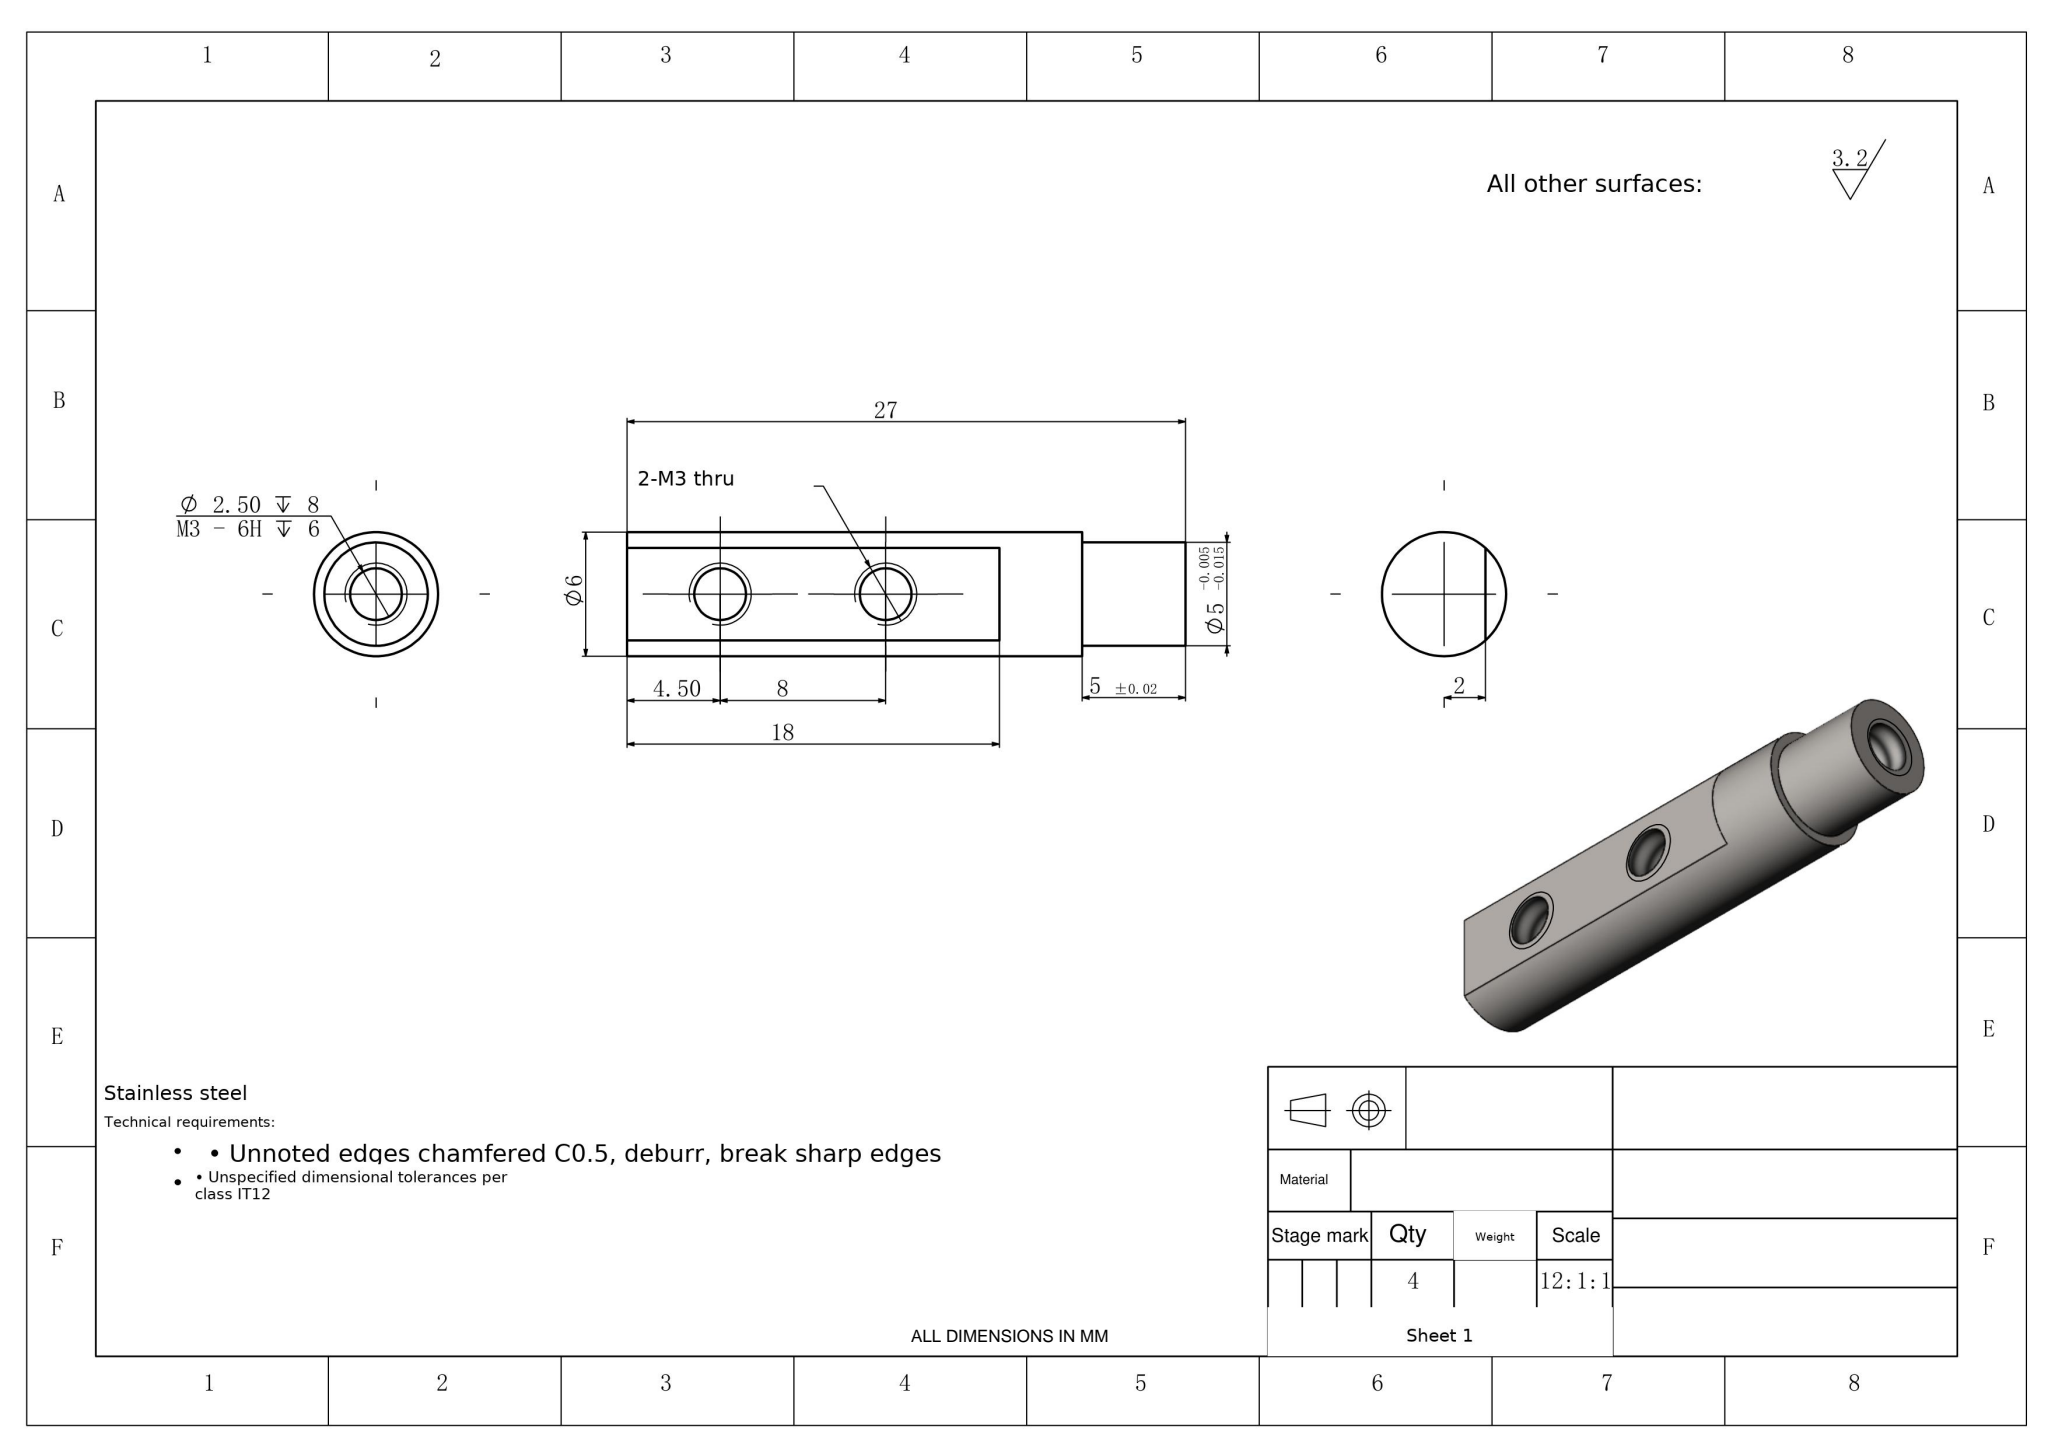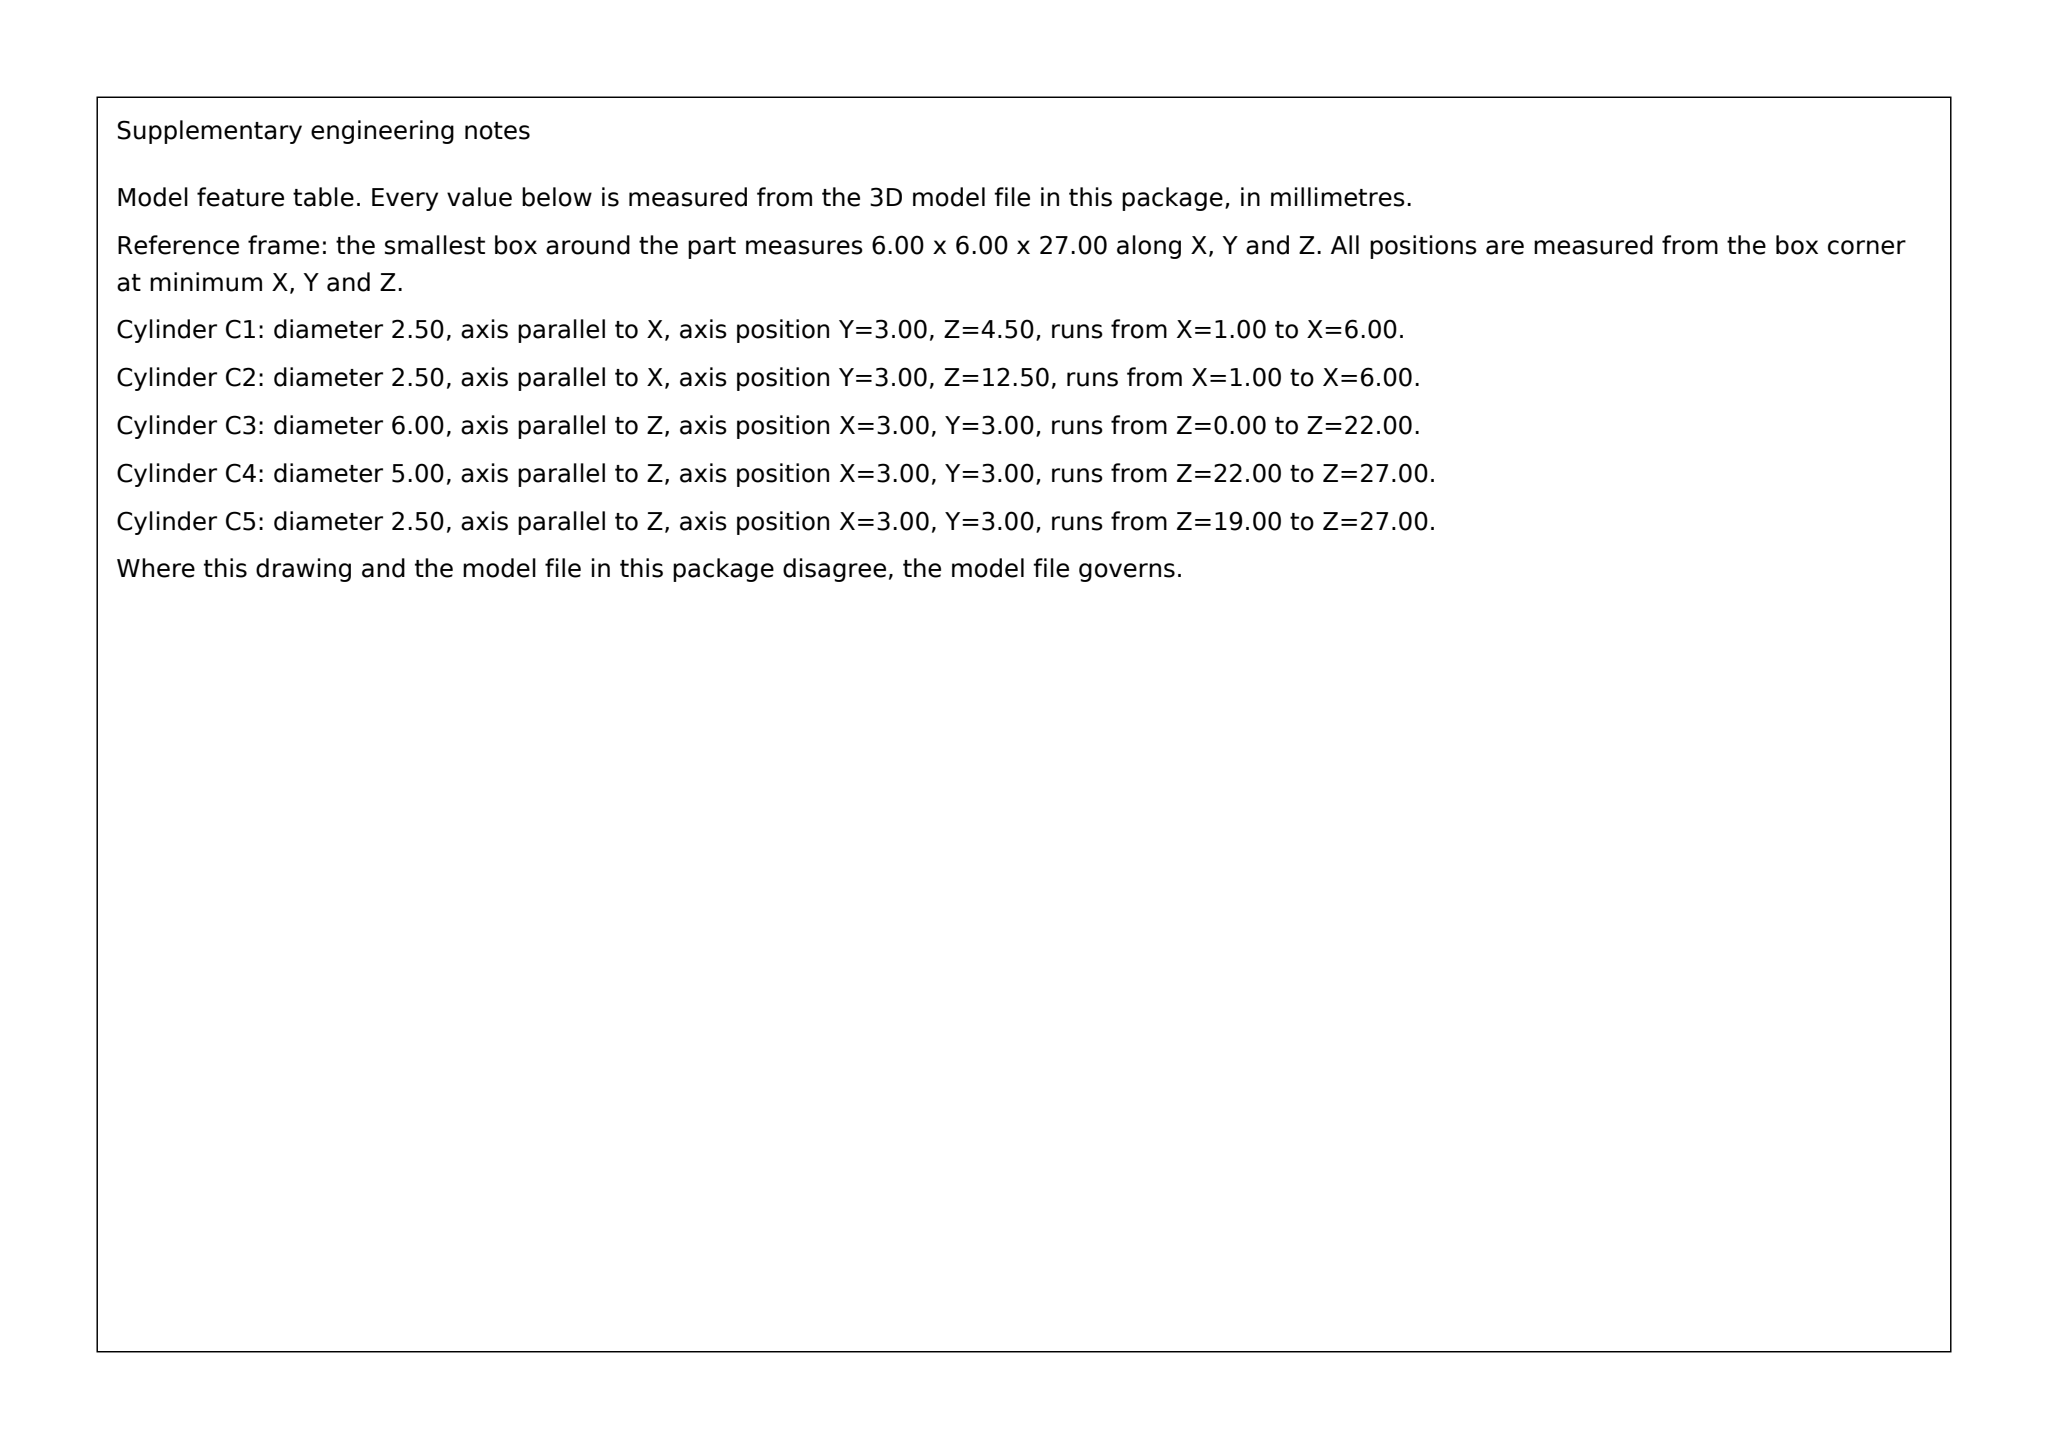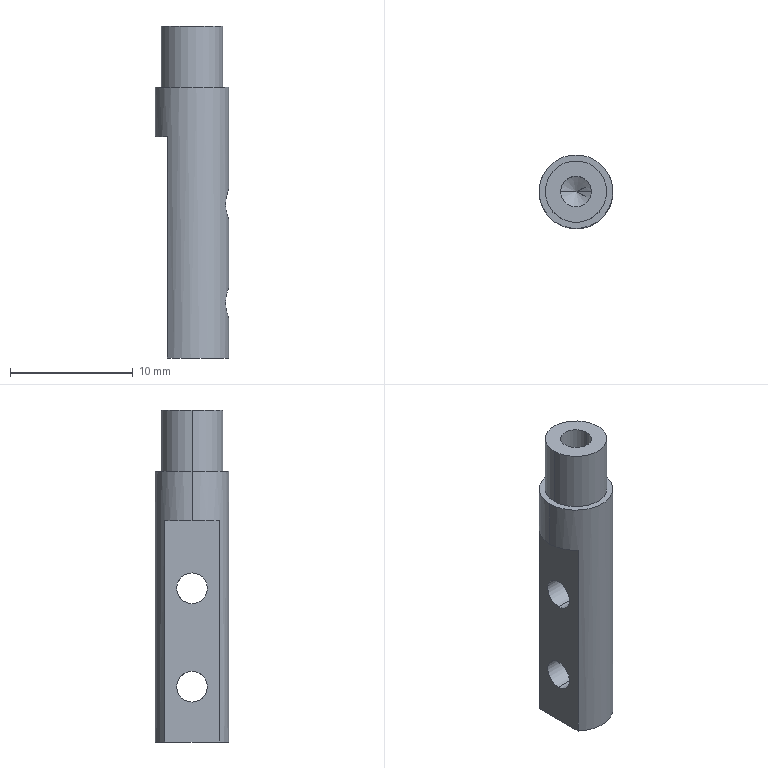Part | SolidWorks | mm | material Stainless steel | 1 solid | 17 faces | box 6 x 6 x 27 mm | volume 576 mm3 | cylinder 10 | plane 5 | cone 2 | commonest cylinder face diameters 2.5 x6 6 x2 5 x2
build123d program:
from build123d import *

# Parameters (mm, degrees)
SKETCH1_R             = 3
BOSS_EXTRUDE1_DEPTH   = 27
SKETCH2_W             = 4.131
SKETCH2_H             = 12.303
CUT_EXTRUDE1_DEPTH    = 18
M3_TAPPED_HOLE3_D     = 2.5
M3_TAPPED_HOLE2_D     = 2.5
M3_TAPPED_HOLE2_DEPTH = 8
M3_TAPPED_HOLE2_TIP   = 0.7511
SKETCH7_R             = 4.398
SKETCH7_R_2           = 2.5
CUT_EXTRUDE2_DEPTH    = 5


with BuildPart() as part:
    # Sketch1 → Boss-Extrude1 (new body)
    with BuildSketch(Plane.XY):
        Circle(SKETCH1_R)
    extrude(amount=BOSS_EXTRUDE1_DEPTH)

    # Sketch2 → Cut-Extrude1 (cut)
    with BuildSketch(Plane(origin=(0, 0, 0), x_dir=(-1, 0, 0), z_dir=(0, 0, -1))):
        with Locations((4.065, -2.134)):
            Rectangle(SKETCH2_W, SKETCH2_H)
    extrude(amount=-CUT_EXTRUDE1_DEPTH, mode=Mode.SUBTRACT)

    # M3 Tapped Hole3 (through all)
    with Locations(Plane.ZY.offset(2)):
        with Locations((12.5, 0), (4.5, 0)):
            Hole(M3_TAPPED_HOLE3_D / 2)

    # M3 Tapped Hole2
    with Locations(Plane.XY.offset(27)):
        with Locations((0, 0)):
            Hole(M3_TAPPED_HOLE2_D / 2, depth=M3_TAPPED_HOLE2_DEPTH)
            with Locations((0, 0, -(M3_TAPPED_HOLE2_DEPTH + M3_TAPPED_HOLE2_TIP / 2))):  # 118° drill point
                Cone(0, M3_TAPPED_HOLE2_D / 2, M3_TAPPED_HOLE2_TIP, mode=Mode.SUBTRACT)

    # Sketch7 → Cut-Extrude2 (cut)
    with BuildSketch(Plane.XY.offset(27)):
        Circle(SKETCH7_R)
        Circle(SKETCH7_R_2, mode=Mode.SUBTRACT)
    extrude(amount=-CUT_EXTRUDE2_DEPTH, mode=Mode.SUBTRACT)


solid = part.part
STEP:
#1=CARTESIAN_POINT('',(3.,0.,22.));
#2=VERTEX_POINT('',#1);
#3=CARTESIAN_POINT('',(-3.,0.,22.));
#4=VERTEX_POINT('',#3);
#5=CARTESIAN_POINT('',(0.,0.,22.));
#6=DIRECTION('',(0.,0.,1.));
#7=DIRECTION('',(1.,0.,0.));
#8=AXIS2_PLACEMENT_3D('',#5,#6,#7);
#9=CIRCLE('',#8,3.);
#10=EDGE_CURVE('',#2,#4,#9,.T.);
#11=ORIENTED_EDGE('',*,*,#10,.F.);
#12=CARTESIAN_POINT('',(3.,0.,13.75));
#13=VERTEX_POINT('',#12);
#14=CARTESIAN_POINT('',(3.,0.,27.));
#15=DIRECTION('',(0.,0.,-1.));
#16=VECTOR('',#15,1000.);
#17=LINE('',#14,#16);
#18=EDGE_CURVE('',#2,#13,#17,.T.);
#19=ORIENTED_EDGE('',*,*,#18,.T.);
#20=CARTESIAN_POINT('',(3.,0.,11.25));
#21=VERTEX_POINT('',#20);
#22=CARTESIAN_POINT('',(3.,0.,13.75));
#23=CARTESIAN_POINT('',(3.,0.08362,13.75));
#24=CARTESIAN_POINT('',(2.997,0.1657,13.742));
#25=CARTESIAN_POINT('',(2.983,0.3268,13.709));
#26=CARTESIAN_POINT('',(2.973,0.4067,13.685));
#27=CARTESIAN_POINT('',(2.936,0.6333,13.59));
#28=CARTESIAN_POINT('',(2.902,0.7706,13.497));
#29=CARTESIAN_POINT('',(2.832,0.9984,13.269));
#30=CARTESIAN_POINT('',(2.795,1.091,13.132));
#31=CARTESIAN_POINT('',(2.743,1.216,12.832));
#32=CARTESIAN_POINT('',(2.727,1.25,12.666));
#33=CARTESIAN_POINT('',(2.727,1.25,12.418));
#34=CARTESIAN_POINT('',(2.731,1.242,12.334));
#35=CARTESIAN_POINT('',(2.746,1.209,12.173));
#36=CARTESIAN_POINT('',(2.756,1.185,12.094));
#37=CARTESIAN_POINT('',(2.796,1.09,11.866));
#38=CARTESIAN_POINT('',(2.832,0.9979,11.73));
#39=CARTESIAN_POINT('',(2.902,0.7693,11.502));
#40=CARTESIAN_POINT('',(2.937,0.6315,11.409));
#41=CARTESIAN_POINT('',(2.986,0.3311,11.284));
#42=CARTESIAN_POINT('',(3.,0.1647,11.25));
#43=CARTESIAN_POINT('',(3.,0.,11.25));
#44=B_SPLINE_CURVE_WITH_KNOTS('',3,(#22,#23,#24,#25,#26,#27,#28,#29,#30,#31,#32,#33,#34,#35,#36,#37,#38,#39,#40,#41,#42,#43),.UNSPECIFIED.,.F.,.F.,(4,2,2,2,2,2,2,2,2,2,4),(0.,0.0002471,0.0004942,0.0009884,0.001483,0.001977,0.002224,0.002471,0.002965,0.003459,0.003954),.UNSPECIFIED.);
#45=EDGE_CURVE('',#13,#21,#44,.T.);
#46=ORIENTED_EDGE('',*,*,#45,.T.);
#47=CARTESIAN_POINT('',(3.,0.,5.75));
#48=VERTEX_POINT('',#47);
#49=CARTESIAN_POINT('',(3.,0.,27.));
#50=DIRECTION('',(0.,0.,-1.));
#51=VECTOR('',#50,1000.);
#52=LINE('',#49,#51);
#53=EDGE_CURVE('',#21,#48,#52,.T.);
#54=ORIENTED_EDGE('',*,*,#53,.T.);
#55=CARTESIAN_POINT('',(3.,0.,3.25));
#56=VERTEX_POINT('',#55);
#57=CARTESIAN_POINT('',(3.,0.,5.75));
#58=CARTESIAN_POINT('',(3.,0.08362,5.75));
#59=CARTESIAN_POINT('',(2.997,0.1657,5.742));
#60=CARTESIAN_POINT('',(2.983,0.3268,5.709));
#61=CARTESIAN_POINT('',(2.973,0.4067,5.685));
#62=CARTESIAN_POINT('',(2.936,0.6333,5.59));
#63=CARTESIAN_POINT('',(2.902,0.7706,5.497));
#64=CARTESIAN_POINT('',(2.832,0.9984,5.269));
#65=CARTESIAN_POINT('',(2.795,1.091,5.132));
#66=CARTESIAN_POINT('',(2.743,1.216,4.832));
#67=CARTESIAN_POINT('',(2.727,1.25,4.666));
#68=CARTESIAN_POINT('',(2.727,1.25,4.418));
#69=CARTESIAN_POINT('',(2.731,1.242,4.334));
#70=CARTESIAN_POINT('',(2.746,1.209,4.173));
#71=CARTESIAN_POINT('',(2.756,1.185,4.094));
#72=CARTESIAN_POINT('',(2.796,1.09,3.866));
#73=CARTESIAN_POINT('',(2.832,0.9979,3.73));
#74=CARTESIAN_POINT('',(2.902,0.7693,3.502));
#75=CARTESIAN_POINT('',(2.937,0.6315,3.409));
#76=CARTESIAN_POINT('',(2.986,0.3311,3.284));
#77=CARTESIAN_POINT('',(3.,0.1647,3.25));
#78=CARTESIAN_POINT('',(3.,0.,3.25));
#79=B_SPLINE_CURVE_WITH_KNOTS('',3,(#57,#58,#59,#60,#61,#62,#63,#64,#65,#66,#67,#68,#69,#70,#71,#72,#73,#74,#75,#76,#77,#78),.UNSPECIFIED.,.F.,.F.,(4,2,2,2,2,2,2,2,2,2,4),(0.,0.0002471,0.0004942,0.0009884,0.001483,0.001977,0.002224,0.002471,0.002965,0.003459,0.003954),.UNSPECIFIED.);
#80=EDGE_CURVE('',#48,#56,#79,.T.);
#81=ORIENTED_EDGE('',*,*,#80,.T.);
#82=CARTESIAN_POINT('',(3.,0.,0.));
#83=VERTEX_POINT('',#82);
#84=CARTESIAN_POINT('',(3.,0.,27.));
#85=DIRECTION('',(0.,0.,-1.));
#86=VECTOR('',#85,1000.);
#87=LINE('',#84,#86);
#88=EDGE_CURVE('',#56,#83,#87,.T.);
#89=ORIENTED_EDGE('',*,*,#88,.T.);
#90=CARTESIAN_POINT('',(-2.,2.236,0.));
#91=VERTEX_POINT('',#90);
#92=CARTESIAN_POINT('',(0.,0.,0.));
#93=DIRECTION('',(0.,0.,1.));
#94=DIRECTION('',(1.,0.,0.));
#95=AXIS2_PLACEMENT_3D('',#92,#93,#94);
#96=CIRCLE('',#95,3.);
#97=EDGE_CURVE('',#83,#91,#96,.T.);
#98=ORIENTED_EDGE('',*,*,#97,.T.);
#99=CARTESIAN_POINT('',(-2.,2.236,18.));
#100=VERTEX_POINT('',#99);
#101=CARTESIAN_POINT('',(-2.,2.236,27.));
#102=DIRECTION('',(0.,0.,1.));
#103=VECTOR('',#102,1000.);
#104=LINE('',#101,#103);
#105=EDGE_CURVE('',#91,#100,#104,.T.);
#106=ORIENTED_EDGE('',*,*,#105,.T.);
#107=CARTESIAN_POINT('',(-3.,0.,18.));
#108=VERTEX_POINT('',#107);
#109=CARTESIAN_POINT('',(0.,0.,18.));
#110=DIRECTION('',(0.,0.,1.));
#111=DIRECTION('',(1.,0.,0.));
#112=AXIS2_PLACEMENT_3D('',#109,#110,#111);
#113=CIRCLE('',#112,3.);
#114=EDGE_CURVE('',#100,#108,#113,.T.);
#115=ORIENTED_EDGE('',*,*,#114,.T.);
#116=CARTESIAN_POINT('',(-3.,0.,27.));
#117=DIRECTION('',(0.,0.,-1.));
#118=VECTOR('',#117,1000.);
#119=LINE('',#116,#118);
#120=EDGE_CURVE('',#4,#108,#119,.T.);
#121=ORIENTED_EDGE('',*,*,#120,.F.);
#122=EDGE_LOOP('',(#11,#19,#46,#54,#81,#89,#98,#106,#115,#121));
#123=FACE_OUTER_BOUND('',#122,.T.);
#124=CARTESIAN_POINT('',(0.,0.,27.));
#125=DIRECTION('',(0.,0.,-1.));
#126=DIRECTION('',(-1.,0.,0.));
#127=AXIS2_PLACEMENT_3D('',#124,#125,#126);
#128=CYLINDRICAL_SURFACE('',#127,3.);
#129=ADVANCED_FACE('',(#123),#128,.T.);
#130=CARTESIAN_POINT('',(3.,0.,3.25));
#131=CARTESIAN_POINT('',(3.,-0.1646,3.25));
#132=CARTESIAN_POINT('',(2.986,-0.3304,3.283));
#133=CARTESIAN_POINT('',(2.936,-0.6331,3.41));
#134=CARTESIAN_POINT('',(2.902,-0.7697,3.502));
#135=CARTESIAN_POINT('',(2.849,-0.9421,3.674));
#136=CARTESIAN_POINT('',(2.831,-0.9932,3.737));
#137=CARTESIAN_POINT('',(2.798,-1.083,3.871));
#138=CARTESIAN_POINT('',(2.782,-1.122,3.944));
#139=CARTESIAN_POINT('',(2.756,-1.185,4.094));
#140=CARTESIAN_POINT('',(2.746,-1.209,4.172));
#141=CARTESIAN_POINT('',(2.731,-1.242,4.333));
#142=CARTESIAN_POINT('',(2.727,-1.25,4.417));
#143=CARTESIAN_POINT('',(2.727,-1.25,4.664));
#144=CARTESIAN_POINT('',(2.743,-1.217,4.83));
#145=CARTESIAN_POINT('',(2.795,-1.091,5.132));
#146=CARTESIAN_POINT('',(2.831,-0.9991,5.269));
#147=CARTESIAN_POINT('',(2.902,-0.7697,5.498));
#148=CARTESIAN_POINT('',(2.936,-0.6344,5.59));
#149=CARTESIAN_POINT('',(2.986,-0.3296,5.717));
#150=CARTESIAN_POINT('',(3.,-0.1671,5.75));
#151=CARTESIAN_POINT('',(3.,0.,5.75));
#152=B_SPLINE_CURVE_WITH_KNOTS('',3,(#130,#131,#132,#133,#134,#135,#136,#137,#138,#139,#140,#141,#142,#143,#144,#145,#146,#147,#148,#149,#150,#151),.UNSPECIFIED.,.F.,.F.,(4,2,2,2,2,2,2,2,2,2,4),(0.003954,0.004448,0.004941,0.005188,0.005435,0.005682,0.005929,0.006423,0.006917,0.00741,0.007904),.UNSPECIFIED.);
#153=EDGE_CURVE('',#56,#48,#152,.T.);
#154=ORIENTED_EDGE('',*,*,#153,.F.);
#155=CARTESIAN_POINT('',(-2.,0.,3.25));
#156=VERTEX_POINT('',#155);
#157=CARTESIAN_POINT('',(-2.,0.,3.25));
#158=DIRECTION('',(-1.,0.,0.));
#159=VECTOR('',#158,1000.);
#160=LINE('',#157,#159);
#161=EDGE_CURVE('',#56,#156,#160,.T.);
#162=ORIENTED_EDGE('',*,*,#161,.T.);
#163=CARTESIAN_POINT('',(-2.,0.,5.75));
#164=VERTEX_POINT('',#163);
#165=CARTESIAN_POINT('',(-2.,0.,4.5));
#166=DIRECTION('',(-1.,0.,0.));
#167=DIRECTION('',(0.,0.,1.));
#168=AXIS2_PLACEMENT_3D('',#165,#166,#167);
#169=CIRCLE('',#168,1.25);
#170=EDGE_CURVE('',#156,#164,#169,.T.);
#171=ORIENTED_EDGE('',*,*,#170,.T.);
#172=CARTESIAN_POINT('',(-2.,0.,5.75));
#173=DIRECTION('',(-1.,0.,0.));
#174=VECTOR('',#173,1000.);
#175=LINE('',#172,#174);
#176=EDGE_CURVE('',#48,#164,#175,.T.);
#177=ORIENTED_EDGE('',*,*,#176,.F.);
#178=EDGE_LOOP('',(#154,#162,#171,#177));
#179=FACE_OUTER_BOUND('',#178,.T.);
#180=CARTESIAN_POINT('',(-2.,0.,4.5));
#181=DIRECTION('',(-1.,0.,0.));
#182=DIRECTION('',(0.,0.,1.));
#183=AXIS2_PLACEMENT_3D('',#180,#181,#182);
#184=CYLINDRICAL_SURFACE('',#183,1.25);
#185=ADVANCED_FACE('',(#179),#184,.F.);
#186=CARTESIAN_POINT('',(3.,0.,11.25));
#187=CARTESIAN_POINT('',(3.,-0.1646,11.25));
#188=CARTESIAN_POINT('',(2.986,-0.3304,11.283));
#189=CARTESIAN_POINT('',(2.936,-0.6331,11.41));
#190=CARTESIAN_POINT('',(2.902,-0.7697,11.502));
#191=CARTESIAN_POINT('',(2.849,-0.9421,11.674));
#192=CARTESIAN_POINT('',(2.831,-0.9932,11.737));
#193=CARTESIAN_POINT('',(2.798,-1.083,11.871));
#194=CARTESIAN_POINT('',(2.782,-1.122,11.944));
#195=CARTESIAN_POINT('',(2.756,-1.185,12.094));
#196=CARTESIAN_POINT('',(2.746,-1.209,12.172));
#197=CARTESIAN_POINT('',(2.731,-1.242,12.333));
#198=CARTESIAN_POINT('',(2.727,-1.25,12.417));
#199=CARTESIAN_POINT('',(2.727,-1.25,12.664));
#200=CARTESIAN_POINT('',(2.743,-1.217,12.83));
#201=CARTESIAN_POINT('',(2.795,-1.091,13.132));
#202=CARTESIAN_POINT('',(2.831,-0.9991,13.269));
#203=CARTESIAN_POINT('',(2.902,-0.7697,13.498));
#204=CARTESIAN_POINT('',(2.936,-0.6344,13.59));
#205=CARTESIAN_POINT('',(2.986,-0.3296,13.717));
#206=CARTESIAN_POINT('',(3.,-0.1671,13.75));
#207=CARTESIAN_POINT('',(3.,0.,13.75));
#208=B_SPLINE_CURVE_WITH_KNOTS('',3,(#186,#187,#188,#189,#190,#191,#192,#193,#194,#195,#196,#197,#198,#199,#200,#201,#202,#203,#204,#205,#206,#207),.UNSPECIFIED.,.F.,.F.,(4,2,2,2,2,2,2,2,2,2,4),(0.003954,0.004448,0.004941,0.005188,0.005435,0.005682,0.005929,0.006423,0.006917,0.00741,0.007904),.UNSPECIFIED.);
#209=EDGE_CURVE('',#21,#13,#208,.T.);
#210=ORIENTED_EDGE('',*,*,#209,.F.);
#211=CARTESIAN_POINT('',(-2.,0.,11.25));
#212=VERTEX_POINT('',#211);
#213=CARTESIAN_POINT('',(-2.,0.,11.25));
#214=DIRECTION('',(-1.,0.,0.));
#215=VECTOR('',#214,1000.);
#216=LINE('',#213,#215);
#217=EDGE_CURVE('',#21,#212,#216,.T.);
#218=ORIENTED_EDGE('',*,*,#217,.T.);
#219=CARTESIAN_POINT('',(-2.,0.,13.75));
#220=VERTEX_POINT('',#219);
#221=CARTESIAN_POINT('',(-2.,0.,12.5));
#222=DIRECTION('',(-1.,0.,0.));
#223=DIRECTION('',(0.,0.,1.));
#224=AXIS2_PLACEMENT_3D('',#221,#222,#223);
#225=CIRCLE('',#224,1.25);
#226=EDGE_CURVE('',#212,#220,#225,.T.);
#227=ORIENTED_EDGE('',*,*,#226,.T.);
#228=CARTESIAN_POINT('',(-2.,0.,13.75));
#229=DIRECTION('',(-1.,0.,0.));
#230=VECTOR('',#229,1000.);
#231=LINE('',#228,#230);
#232=EDGE_CURVE('',#13,#220,#231,.T.);
#233=ORIENTED_EDGE('',*,*,#232,.F.);
#234=EDGE_LOOP('',(#210,#218,#227,#233));
#235=FACE_OUTER_BOUND('',#234,.T.);
#236=CARTESIAN_POINT('',(-2.,0.,12.5));
#237=DIRECTION('',(-1.,0.,0.));
#238=DIRECTION('',(0.,0.,1.));
#239=AXIS2_PLACEMENT_3D('',#236,#237,#238);
#240=CYLINDRICAL_SURFACE('',#239,1.25);
#241=ADVANCED_FACE('',(#235),#240,.F.);
#242=CARTESIAN_POINT('',(2.5,0.,22.));
#243=VERTEX_POINT('',#242);
#244=CARTESIAN_POINT('',(-2.5,0.,22.));
#245=VERTEX_POINT('',#244);
#246=CARTESIAN_POINT('',(0.,0.,22.));
#247=DIRECTION('',(0.,0.,1.));
#248=DIRECTION('',(1.,0.,0.));
#249=AXIS2_PLACEMENT_3D('',#246,#247,#248);
#250=CIRCLE('',#249,2.5);
#251=EDGE_CURVE('',#243,#245,#250,.T.);
#252=ORIENTED_EDGE('',*,*,#251,.T.);
#253=CARTESIAN_POINT('',(-2.5,0.,27.));
#254=VERTEX_POINT('',#253);
#255=CARTESIAN_POINT('',(-2.5,0.,22.));
#256=DIRECTION('',(0.,0.,1.));
#257=VECTOR('',#256,1000.);
#258=LINE('',#255,#257);
#259=EDGE_CURVE('',#245,#254,#258,.T.);
#260=ORIENTED_EDGE('',*,*,#259,.T.);
#261=CARTESIAN_POINT('',(2.5,0.,27.));
#262=VERTEX_POINT('',#261);
#263=CARTESIAN_POINT('',(0.,0.,27.));
#264=DIRECTION('',(0.,0.,1.));
#265=DIRECTION('',(1.,0.,0.));
#266=AXIS2_PLACEMENT_3D('',#263,#264,#265);
#267=CIRCLE('',#266,2.5);
#268=EDGE_CURVE('',#262,#254,#267,.T.);
#269=ORIENTED_EDGE('',*,*,#268,.F.);
#270=CARTESIAN_POINT('',(2.5,0.,22.));
#271=DIRECTION('',(0.,0.,1.));
#272=VECTOR('',#271,1000.);
#273=LINE('',#270,#272);
#274=EDGE_CURVE('',#243,#262,#273,.T.);
#275=ORIENTED_EDGE('',*,*,#274,.F.);
#276=EDGE_LOOP('',(#252,#260,#269,#275));
#277=FACE_OUTER_BOUND('',#276,.T.);
#278=CARTESIAN_POINT('',(0.,0.,22.));
#279=DIRECTION('',(0.,0.,1.));
#280=DIRECTION('',(1.,0.,0.));
#281=AXIS2_PLACEMENT_3D('',#278,#279,#280);
#282=CYLINDRICAL_SURFACE('',#281,2.5);
#283=ADVANCED_FACE('',(#277),#282,.T.);
#284=CARTESIAN_POINT('',(-1.25,0.,19.));
#285=VERTEX_POINT('',#284);
#286=CARTESIAN_POINT('',(1.25,0.,19.));
#287=VERTEX_POINT('',#286);
#288=CARTESIAN_POINT('',(0.,0.,19.));
#289=DIRECTION('',(0.,0.,1.));
#290=DIRECTION('',(1.,0.,0.));
#291=AXIS2_PLACEMENT_3D('',#288,#289,#290);
#292=CIRCLE('',#291,1.25);
#293=EDGE_CURVE('',#285,#287,#292,.T.);
#294=ORIENTED_EDGE('',*,*,#293,.F.);
#295=CARTESIAN_POINT('',(-1.25,0.,27.));
#296=VERTEX_POINT('',#295);
#297=CARTESIAN_POINT('',(-1.25,0.,27.));
#298=DIRECTION('',(0.,0.,1.));
#299=VECTOR('',#298,1000.);
#300=LINE('',#297,#299);
#301=EDGE_CURVE('',#285,#296,#300,.T.);
#302=ORIENTED_EDGE('',*,*,#301,.T.);
#303=CARTESIAN_POINT('',(1.25,0.,27.));
#304=VERTEX_POINT('',#303);
#305=CARTESIAN_POINT('',(0.,0.,27.));
#306=DIRECTION('',(0.,0.,1.));
#307=DIRECTION('',(1.,0.,0.));
#308=AXIS2_PLACEMENT_3D('',#305,#306,#307);
#309=CIRCLE('',#308,1.25);
#310=EDGE_CURVE('',#296,#304,#309,.T.);
#311=ORIENTED_EDGE('',*,*,#310,.T.);
#312=CARTESIAN_POINT('',(1.25,0.,27.));
#313=DIRECTION('',(0.,0.,1.));
#314=VECTOR('',#313,1000.);
#315=LINE('',#312,#314);
#316=EDGE_CURVE('',#287,#304,#315,.T.);
#317=ORIENTED_EDGE('',*,*,#316,.F.);
#318=EDGE_LOOP('',(#294,#302,#311,#317));
#319=FACE_OUTER_BOUND('',#318,.T.);
#320=CARTESIAN_POINT('',(0.,0.,27.));
#321=DIRECTION('',(0.,0.,1.));
#322=DIRECTION('',(1.,0.,0.));
#323=AXIS2_PLACEMENT_3D('',#320,#321,#322);
#324=CYLINDRICAL_SURFACE('',#323,1.25);
#325=ADVANCED_FACE('',(#319),#324,.F.);
#326=CARTESIAN_POINT('',(-0.,0.,18.249));
#327=VERTEX_POINT('',#326);
#328=CARTESIAN_POINT('',(1.25,0.,19.));
#329=DIRECTION('',(0.8572,0.,0.515));
#330=VECTOR('',#329,1000.);
#331=LINE('',#328,#330);
#332=EDGE_CURVE('',#327,#287,#331,.T.);
#333=ORIENTED_EDGE('',*,*,#332,.F.);
#334=CARTESIAN_POINT('',(-1.25,0.,19.));
#335=DIRECTION('',(-0.8572,0.,0.515));
#336=VECTOR('',#335,1000.);
#337=LINE('',#334,#336);
#338=EDGE_CURVE('',#327,#285,#337,.T.);
#339=ORIENTED_EDGE('',*,*,#338,.T.);
#340=ORIENTED_EDGE('',*,*,#293,.T.);
#341=EDGE_LOOP('',(#333,#339,#340));
#342=FACE_OUTER_BOUND('',#341,.T.);
#343=CARTESIAN_POINT('',(0.,0.,19.));
#344=DIRECTION('',(0.,0.,1.));
#345=DIRECTION('',(1.,0.,0.));
#346=AXIS2_PLACEMENT_3D('',#343,#344,#345);
#347=CONICAL_SURFACE('',#346,1.25,1.03);
#348=ADVANCED_FACE('',(#342),#347,.F.);
#349=CARTESIAN_POINT('',(0.,0.,27.));
#350=DIRECTION('',(0.,0.,1.));
#351=DIRECTION('',(1.,0.,0.));
#352=AXIS2_PLACEMENT_3D('',#349,#350,#351);
#353=CIRCLE('',#352,1.25);
#354=EDGE_CURVE('',#304,#296,#353,.T.);
#355=ORIENTED_EDGE('',*,*,#354,.F.);
#356=ORIENTED_EDGE('',*,*,#310,.F.);
#357=EDGE_LOOP('',(#355,#356));
#358=FACE_BOUND('',#357,.T.);
#359=ORIENTED_EDGE('',*,*,#268,.T.);
#360=CARTESIAN_POINT('',(0.,0.,27.));
#361=DIRECTION('',(0.,0.,1.));
#362=DIRECTION('',(1.,0.,0.));
#363=AXIS2_PLACEMENT_3D('',#360,#361,#362);
#364=CIRCLE('',#363,2.5);
#365=EDGE_CURVE('',#254,#262,#364,.T.);
#366=ORIENTED_EDGE('',*,*,#365,.T.);
#367=EDGE_LOOP('',(#359,#366));
#368=FACE_OUTER_BOUND('',#367,.T.);
#369=CARTESIAN_POINT('',(0.,0.,27.));
#370=DIRECTION('',(0.,0.,1.));
#371=DIRECTION('',(1.,0.,0.));
#372=AXIS2_PLACEMENT_3D('',#369,#370,#371);
#373=PLANE('',#372);
#374=ADVANCED_FACE('',(#358,#368),#373,.T.);
#375=ORIENTED_EDGE('',*,*,#338,.F.);
#376=ORIENTED_EDGE('',*,*,#332,.T.);
#377=CARTESIAN_POINT('',(0.,0.,19.));
#378=DIRECTION('',(0.,0.,1.));
#379=DIRECTION('',(1.,0.,0.));
#380=AXIS2_PLACEMENT_3D('',#377,#378,#379);
#381=CIRCLE('',#380,1.25);
#382=EDGE_CURVE('',#287,#285,#381,.T.);
#383=ORIENTED_EDGE('',*,*,#382,.T.);
#384=EDGE_LOOP('',(#375,#376,#383));
#385=FACE_OUTER_BOUND('',#384,.T.);
#386=CARTESIAN_POINT('',(0.,0.,19.));
#387=DIRECTION('',(0.,0.,1.));
#388=DIRECTION('',(1.,0.,0.));
#389=AXIS2_PLACEMENT_3D('',#386,#387,#388);
#390=CONICAL_SURFACE('',#389,1.25,1.03);
#391=ADVANCED_FACE('',(#385),#390,.F.);
#392=ORIENTED_EDGE('',*,*,#301,.F.);
#393=ORIENTED_EDGE('',*,*,#382,.F.);
#394=ORIENTED_EDGE('',*,*,#316,.T.);
#395=ORIENTED_EDGE('',*,*,#354,.T.);
#396=EDGE_LOOP('',(#392,#393,#394,#395));
#397=FACE_OUTER_BOUND('',#396,.T.);
#398=CARTESIAN_POINT('',(0.,0.,27.));
#399=DIRECTION('',(0.,0.,1.));
#400=DIRECTION('',(1.,0.,0.));
#401=AXIS2_PLACEMENT_3D('',#398,#399,#400);
#402=CYLINDRICAL_SURFACE('',#401,1.25);
#403=ADVANCED_FACE('',(#397),#402,.F.);
#404=ORIENTED_EDGE('',*,*,#251,.F.);
#405=CARTESIAN_POINT('',(0.,0.,22.));
#406=DIRECTION('',(0.,0.,1.));
#407=DIRECTION('',(1.,0.,0.));
#408=AXIS2_PLACEMENT_3D('',#405,#406,#407);
#409=CIRCLE('',#408,2.5);
#410=EDGE_CURVE('',#245,#243,#409,.T.);
#411=ORIENTED_EDGE('',*,*,#410,.F.);
#412=EDGE_LOOP('',(#404,#411));
#413=FACE_BOUND('',#412,.T.);
#414=CARTESIAN_POINT('',(0.,0.,22.));
#415=DIRECTION('',(0.,0.,1.));
#416=DIRECTION('',(1.,0.,0.));
#417=AXIS2_PLACEMENT_3D('',#414,#415,#416);
#418=CIRCLE('',#417,3.);
#419=EDGE_CURVE('',#4,#2,#418,.T.);
#420=ORIENTED_EDGE('',*,*,#419,.T.);
#421=ORIENTED_EDGE('',*,*,#10,.T.);
#422=EDGE_LOOP('',(#420,#421));
#423=FACE_OUTER_BOUND('',#422,.T.);
#424=CARTESIAN_POINT('',(0.,0.,22.));
#425=DIRECTION('',(0.,0.,1.));
#426=DIRECTION('',(1.,0.,0.));
#427=AXIS2_PLACEMENT_3D('',#424,#425,#426);
#428=PLANE('',#427);
#429=ADVANCED_FACE('',(#413,#423),#428,.T.);
#430=ORIENTED_EDGE('',*,*,#259,.F.);
#431=ORIENTED_EDGE('',*,*,#410,.T.);
#432=ORIENTED_EDGE('',*,*,#274,.T.);
#433=ORIENTED_EDGE('',*,*,#365,.F.);
#434=EDGE_LOOP('',(#430,#431,#432,#433));
#435=FACE_OUTER_BOUND('',#434,.T.);
#436=CARTESIAN_POINT('',(0.,0.,22.));
#437=DIRECTION('',(0.,0.,1.));
#438=DIRECTION('',(1.,0.,0.));
#439=AXIS2_PLACEMENT_3D('',#436,#437,#438);
#440=CYLINDRICAL_SURFACE('',#439,2.5);
#441=ADVANCED_FACE('',(#435),#440,.T.);
#442=ORIENTED_EDGE('',*,*,#217,.F.);
#443=ORIENTED_EDGE('',*,*,#45,.F.);
#444=ORIENTED_EDGE('',*,*,#232,.T.);
#445=CARTESIAN_POINT('',(-2.,0.,12.5));
#446=DIRECTION('',(-1.,0.,0.));
#447=DIRECTION('',(0.,0.,1.));
#448=AXIS2_PLACEMENT_3D('',#445,#446,#447);
#449=CIRCLE('',#448,1.25);
#450=EDGE_CURVE('',#220,#212,#449,.T.);
#451=ORIENTED_EDGE('',*,*,#450,.T.);
#452=EDGE_LOOP('',(#442,#443,#444,#451));
#453=FACE_OUTER_BOUND('',#452,.T.);
#454=CARTESIAN_POINT('',(-2.,0.,12.5));
#455=DIRECTION('',(-1.,0.,0.));
#456=DIRECTION('',(0.,0.,1.));
#457=AXIS2_PLACEMENT_3D('',#454,#455,#456);
#458=CYLINDRICAL_SURFACE('',#457,1.25);
#459=ADVANCED_FACE('',(#453),#458,.F.);
#460=ORIENTED_EDGE('',*,*,#161,.F.);
#461=ORIENTED_EDGE('',*,*,#80,.F.);
#462=ORIENTED_EDGE('',*,*,#176,.T.);
#463=CARTESIAN_POINT('',(-2.,0.,4.5));
#464=DIRECTION('',(-1.,0.,0.));
#465=DIRECTION('',(0.,0.,1.));
#466=AXIS2_PLACEMENT_3D('',#463,#464,#465);
#467=CIRCLE('',#466,1.25);
#468=EDGE_CURVE('',#164,#156,#467,.T.);
#469=ORIENTED_EDGE('',*,*,#468,.T.);
#470=EDGE_LOOP('',(#460,#461,#462,#469));
#471=FACE_OUTER_BOUND('',#470,.T.);
#472=CARTESIAN_POINT('',(-2.,0.,4.5));
#473=DIRECTION('',(-1.,0.,0.));
#474=DIRECTION('',(0.,0.,1.));
#475=AXIS2_PLACEMENT_3D('',#472,#473,#474);
#476=CYLINDRICAL_SURFACE('',#475,1.25);
#477=ADVANCED_FACE('',(#471),#476,.F.);
#478=CARTESIAN_POINT('',(-2.,-2.236,0.));
#479=VERTEX_POINT('',#478);
#480=CARTESIAN_POINT('',(0.,0.,0.));
#481=DIRECTION('',(0.,0.,1.));
#482=DIRECTION('',(1.,0.,0.));
#483=AXIS2_PLACEMENT_3D('',#480,#481,#482);
#484=CIRCLE('',#483,3.);
#485=EDGE_CURVE('',#479,#83,#484,.T.);
#486=ORIENTED_EDGE('',*,*,#485,.F.);
#487=CARTESIAN_POINT('',(-2.,0.,0.));
#488=DIRECTION('',(0.,1.,0.));
#489=VECTOR('',#488,1000.);
#490=LINE('',#487,#489);
#491=EDGE_CURVE('',#479,#91,#490,.T.);
#492=ORIENTED_EDGE('',*,*,#491,.T.);
#493=ORIENTED_EDGE('',*,*,#97,.F.);
#494=EDGE_LOOP('',(#486,#492,#493));
#495=FACE_OUTER_BOUND('',#494,.T.);
#496=CARTESIAN_POINT('',(0.,0.,0.));
#497=DIRECTION('',(0.,0.,1.));
#498=DIRECTION('',(1.,0.,0.));
#499=AXIS2_PLACEMENT_3D('',#496,#497,#498);
#500=PLANE('',#499);
#501=ADVANCED_FACE('',(#495),#500,.F.);
#502=ORIENTED_EDGE('',*,*,#450,.F.);
#503=ORIENTED_EDGE('',*,*,#226,.F.);
#504=EDGE_LOOP('',(#502,#503));
#505=FACE_BOUND('',#504,.T.);
#506=ORIENTED_EDGE('',*,*,#468,.F.);
#507=ORIENTED_EDGE('',*,*,#170,.F.);
#508=EDGE_LOOP('',(#506,#507));
#509=FACE_BOUND('',#508,.T.);
#510=CARTESIAN_POINT('',(-2.,-2.236,18.));
#511=VERTEX_POINT('',#510);
#512=CARTESIAN_POINT('',(-2.,4.017,18.));
#513=DIRECTION('',(-0.,-1.,0.));
#514=VECTOR('',#513,1000.);
#515=LINE('',#512,#514);
#516=EDGE_CURVE('',#100,#511,#515,.T.);
#517=ORIENTED_EDGE('',*,*,#516,.F.);
#518=ORIENTED_EDGE('',*,*,#105,.F.);
#519=ORIENTED_EDGE('',*,*,#491,.F.);
#520=CARTESIAN_POINT('',(-2.,-2.236,27.));
#521=DIRECTION('',(0.,0.,-1.));
#522=VECTOR('',#521,1000.);
#523=LINE('',#520,#522);
#524=EDGE_CURVE('',#511,#479,#523,.T.);
#525=ORIENTED_EDGE('',*,*,#524,.F.);
#526=EDGE_LOOP('',(#517,#518,#519,#525));
#527=FACE_OUTER_BOUND('',#526,.T.);
#528=CARTESIAN_POINT('',(-2.,4.017,18.));
#529=DIRECTION('',(1.,-0.,0.));
#530=DIRECTION('',(0.,1.,0.));
#531=AXIS2_PLACEMENT_3D('',#528,#529,#530);
#532=PLANE('',#531);
#533=ADVANCED_FACE('',(#505,#509,#527),#532,.F.);
#534=ORIENTED_EDGE('',*,*,#516,.T.);
#535=CARTESIAN_POINT('',(0.,0.,18.));
#536=DIRECTION('',(0.,0.,1.));
#537=DIRECTION('',(1.,0.,0.));
#538=AXIS2_PLACEMENT_3D('',#535,#536,#537);
#539=CIRCLE('',#538,3.);
#540=EDGE_CURVE('',#108,#511,#539,.T.);
#541=ORIENTED_EDGE('',*,*,#540,.F.);
#542=ORIENTED_EDGE('',*,*,#114,.F.);
#543=EDGE_LOOP('',(#534,#541,#542));
#544=FACE_OUTER_BOUND('',#543,.T.);
#545=CARTESIAN_POINT('',(0.,0.,18.));
#546=DIRECTION('',(0.,0.,1.));
#547=DIRECTION('',(1.,0.,0.));
#548=AXIS2_PLACEMENT_3D('',#545,#546,#547);
#549=PLANE('',#548);
#550=ADVANCED_FACE('',(#544),#549,.F.);
#551=ORIENTED_EDGE('',*,*,#18,.F.);
#552=ORIENTED_EDGE('',*,*,#419,.F.);
#553=ORIENTED_EDGE('',*,*,#120,.T.);
#554=ORIENTED_EDGE('',*,*,#540,.T.);
#555=ORIENTED_EDGE('',*,*,#524,.T.);
#556=ORIENTED_EDGE('',*,*,#485,.T.);
#557=ORIENTED_EDGE('',*,*,#88,.F.);
#558=ORIENTED_EDGE('',*,*,#153,.T.);
#559=ORIENTED_EDGE('',*,*,#53,.F.);
#560=ORIENTED_EDGE('',*,*,#209,.T.);
#561=EDGE_LOOP('',(#551,#552,#553,#554,#555,#556,#557,#558,#559,#560));
#562=FACE_OUTER_BOUND('',#561,.T.);
#563=CARTESIAN_POINT('',(0.,0.,27.));
#564=DIRECTION('',(0.,0.,-1.));
#565=DIRECTION('',(-1.,0.,0.));
#566=AXIS2_PLACEMENT_3D('',#563,#564,#565);
#567=CYLINDRICAL_SURFACE('',#566,3.);
#568=ADVANCED_FACE('',(#562),#567,.T.);
#569=CLOSED_SHELL('',(#129,#185,#241,#283,#325,#348,#374,#391,#403,#429,#441,#459,#477,#501,#533,#550,#568));
#570=MANIFOLD_SOLID_BREP('',#569);
#571=CARTESIAN_POINT('',(0.,0.,0.));
#572=DIRECTION('',(0.,0.,1.));
#573=DIRECTION('',(1.,0.,0.));
#574=AXIS2_PLACEMENT_3D('',#571,#572,#573);
#575=(LENGTH_UNIT()NAMED_UNIT(*)SI_UNIT(.MILLI.,.METRE.));
#576=UNCERTAINTY_MEASURE_WITH_UNIT(LENGTH_MEASURE(0.00001),#575,'','');
#577=(NAMED_UNIT(*)PLANE_ANGLE_UNIT()SI_UNIT($,.RADIAN.));
#578=(NAMED_UNIT(*)SI_UNIT($,.STERADIAN.)SOLID_ANGLE_UNIT());
#579=(GEOMETRIC_REPRESENTATION_CONTEXT(3)GLOBAL_UNCERTAINTY_ASSIGNED_CONTEXT((#576))GLOBAL_UNIT_ASSIGNED_CONTEXT((#575,#577,#578))REPRESENTATION_CONTEXT('',''));
#580=ADVANCED_BREP_SHAPE_REPRESENTATION('',(#570,#574),#579);